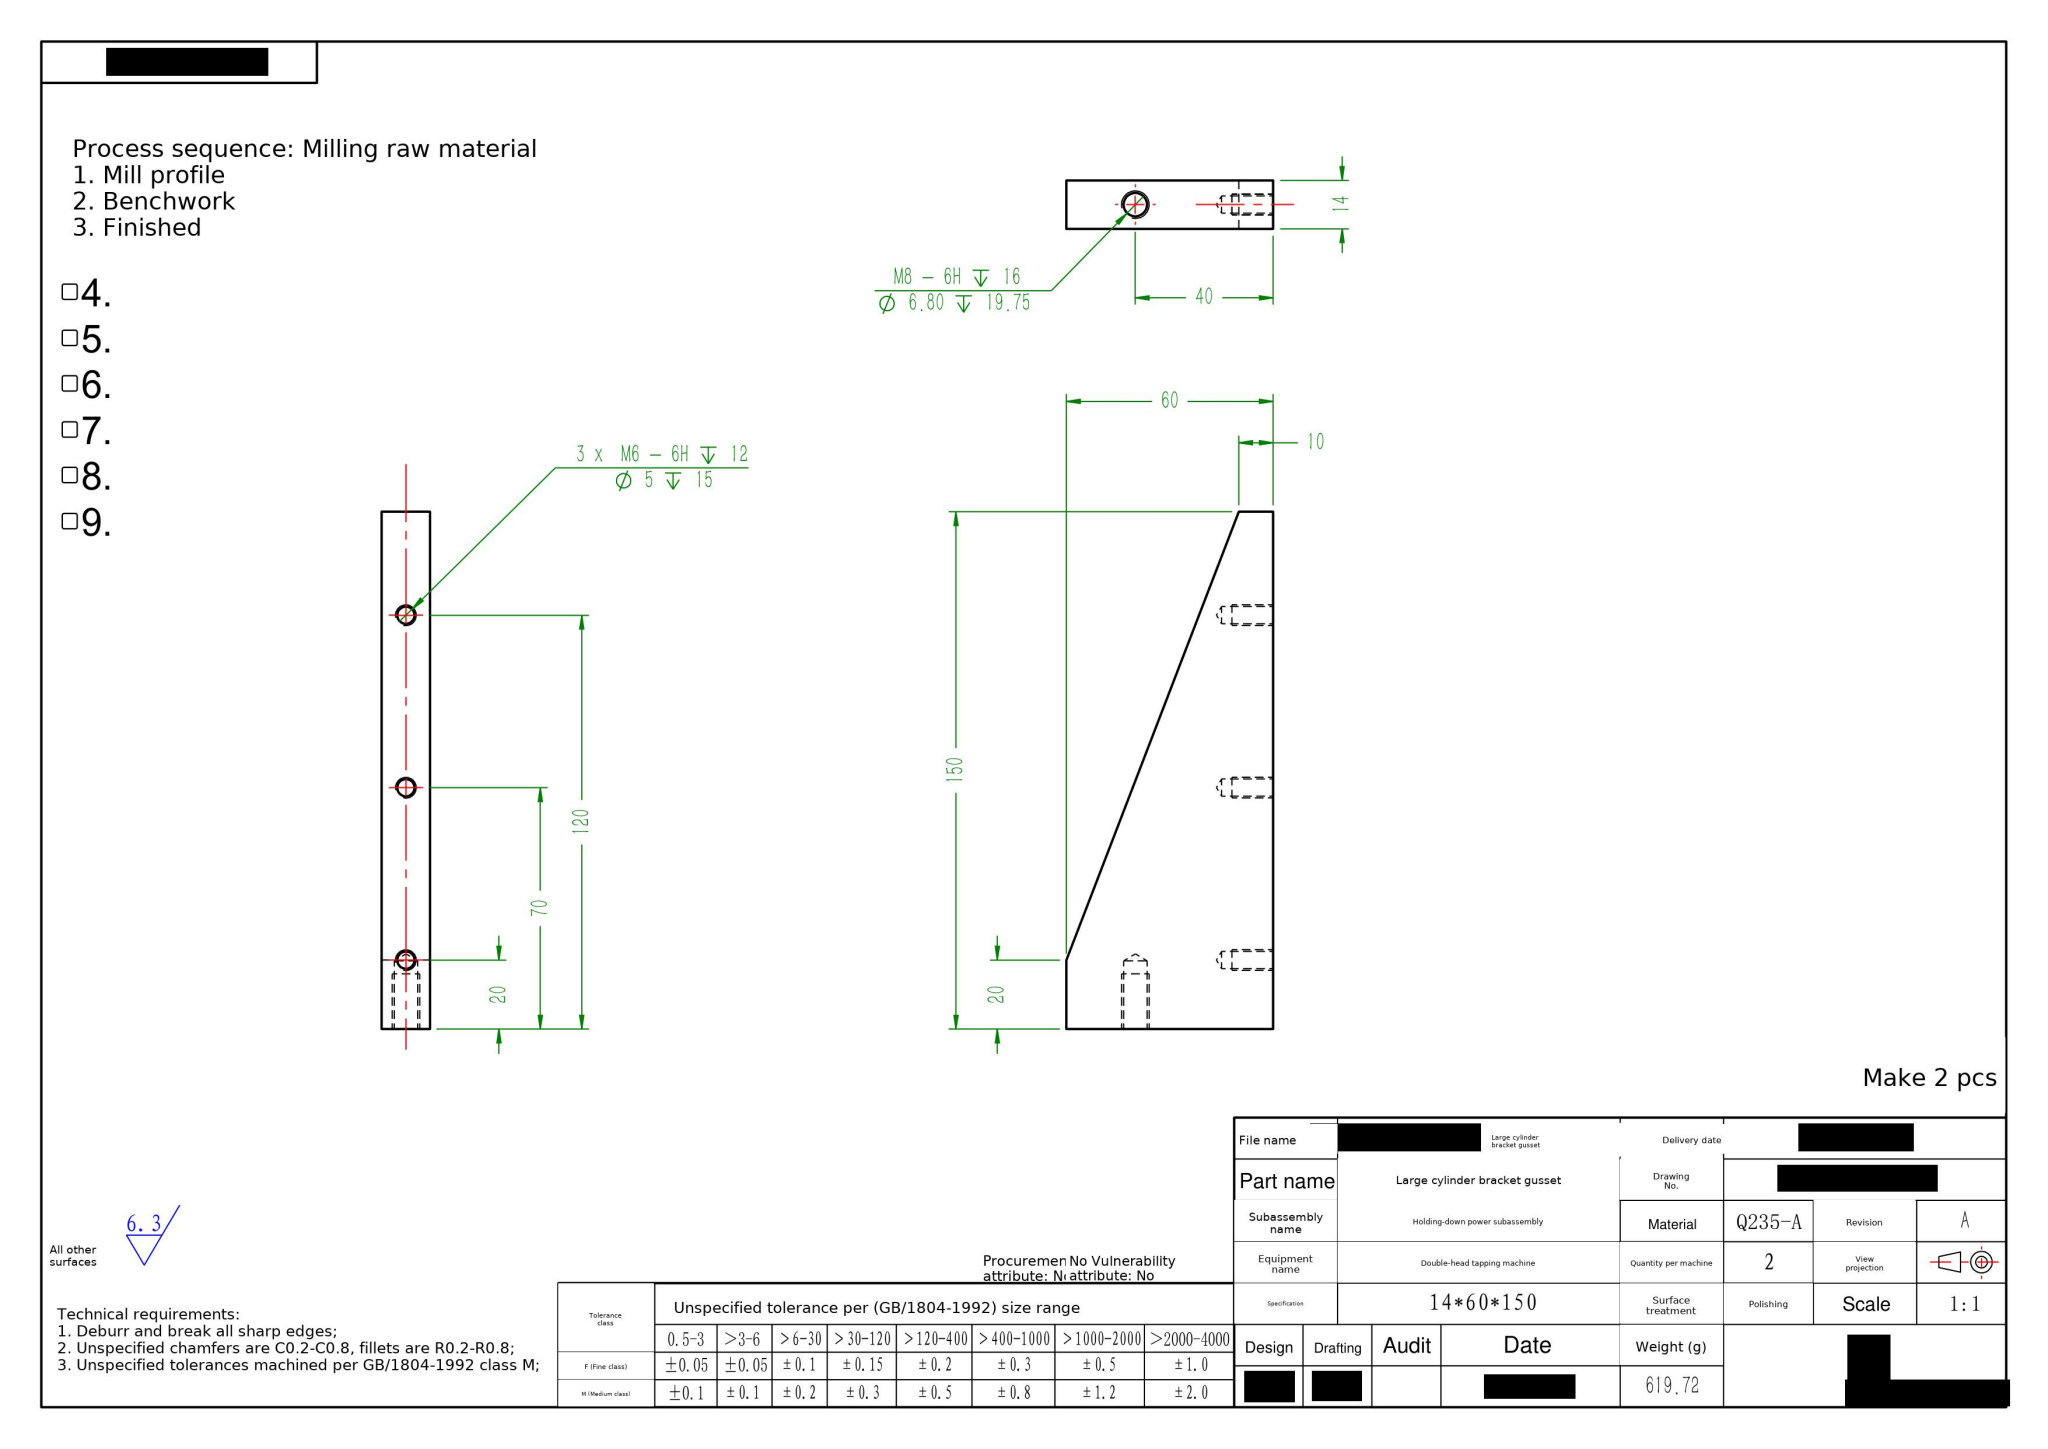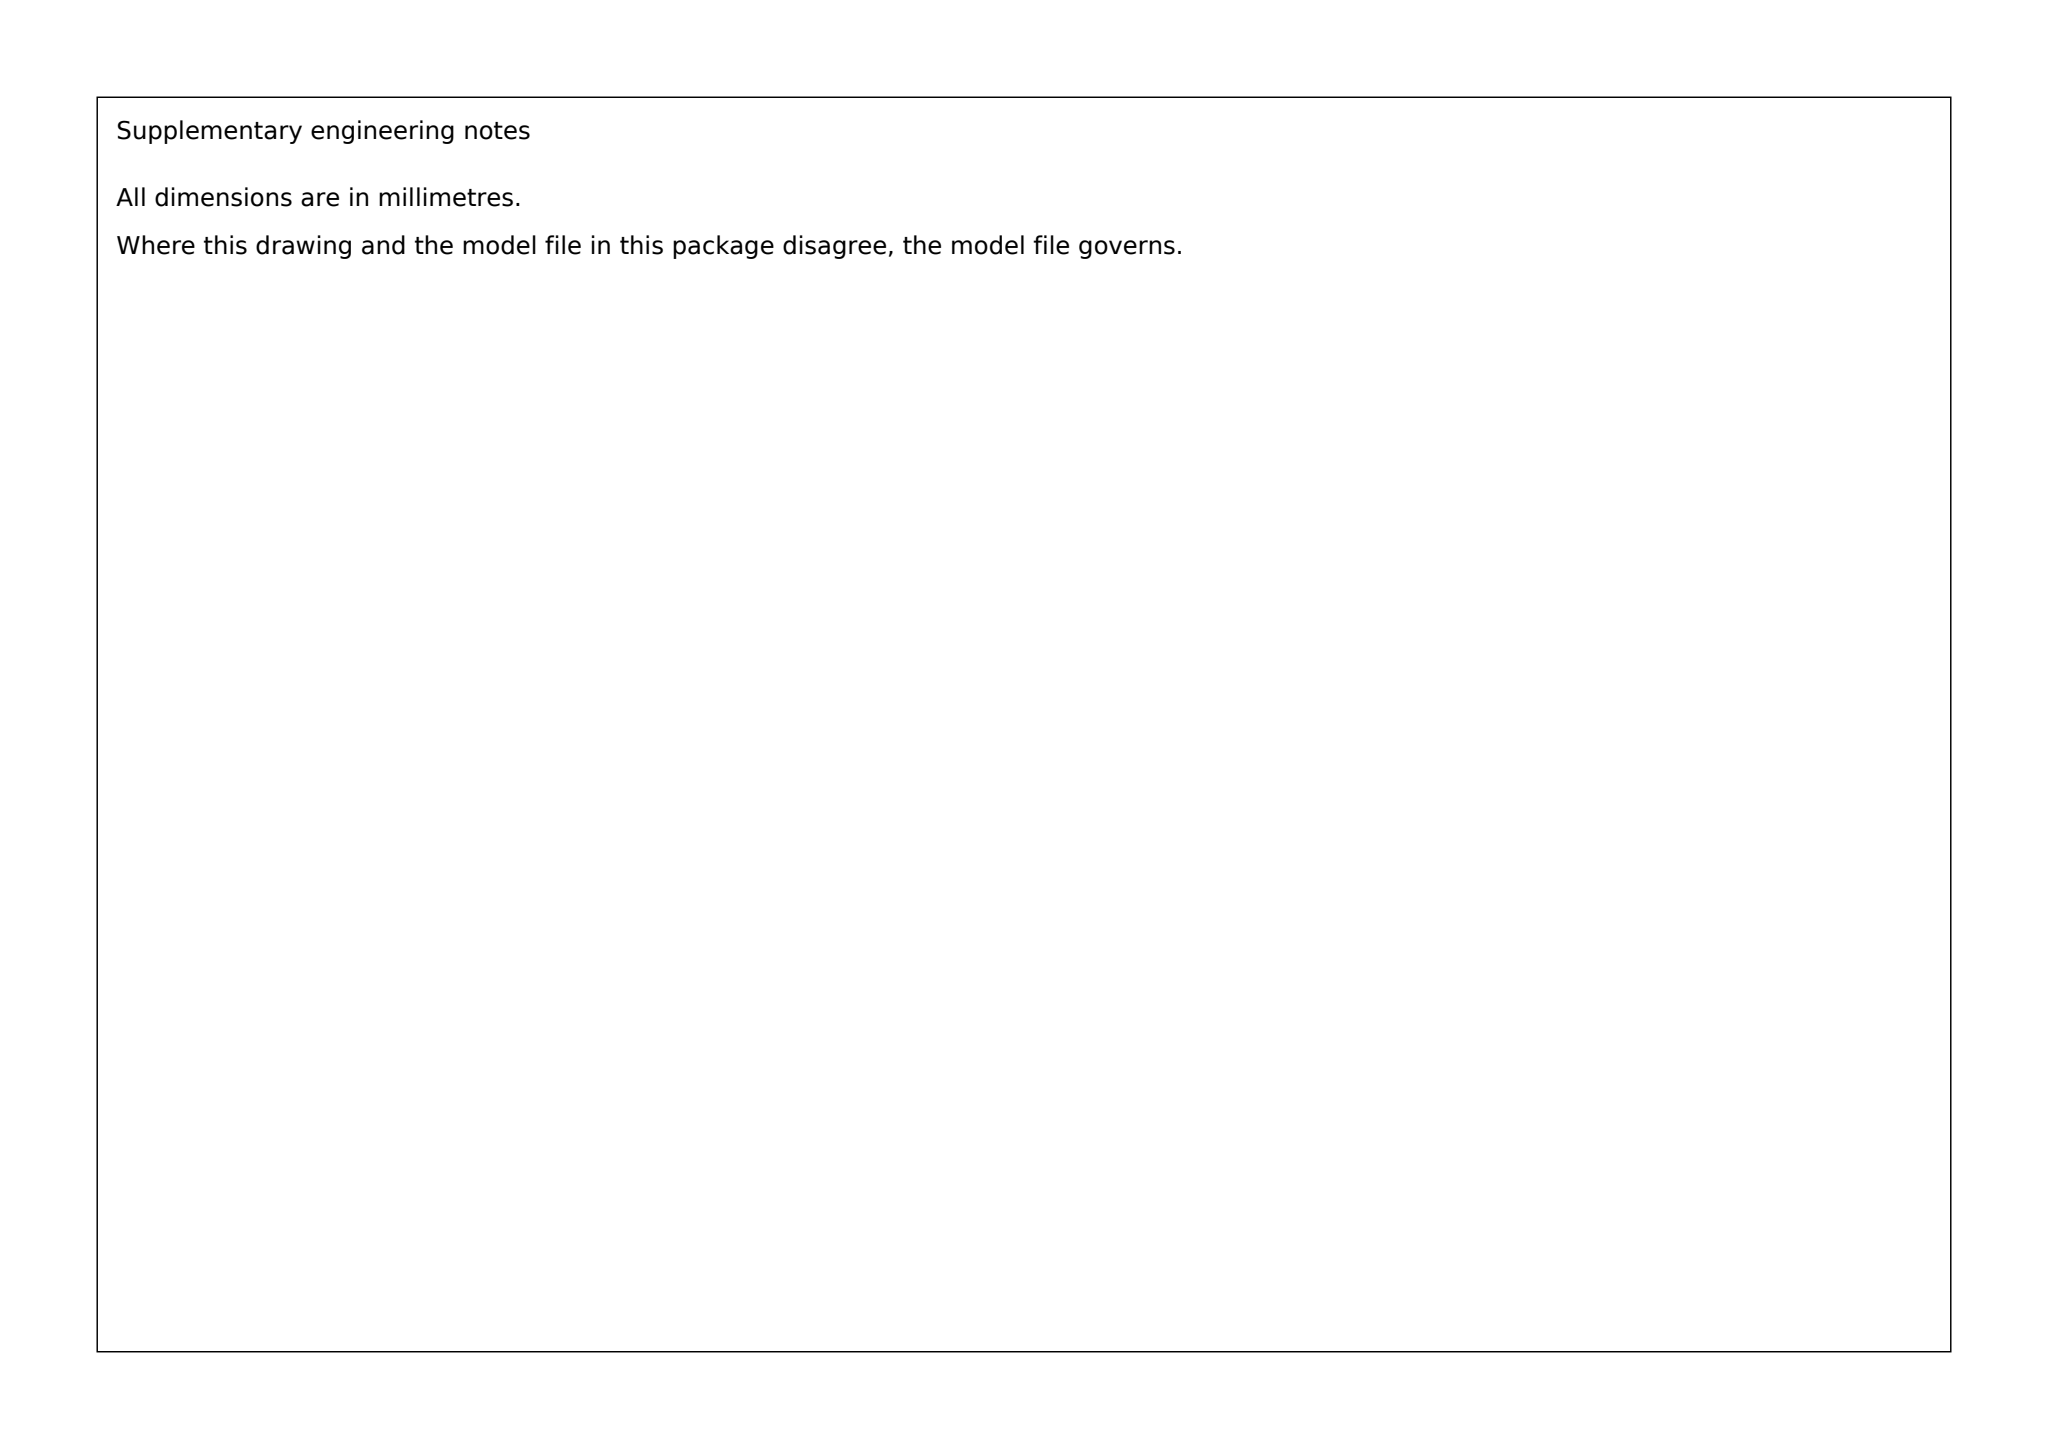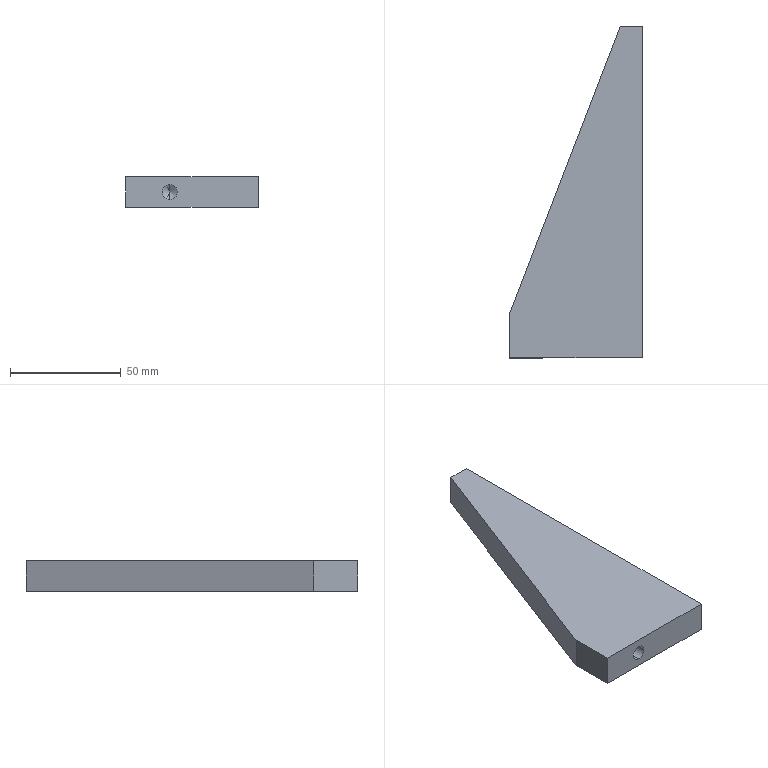Part | SolidWorks | mm | material Q235-A | 1 solid | 23 faces | box 60 x 150 x 14 mm | volume 78845 mm3 | cylinder 8 | cone 8 | plane 7 | commonest cylinder face diameters 5 x6 6.8 x2
build123d program:
from build123d import *

# Parameters (mm, degrees)
BOSS_EXTRUDE1_DEPTH   = 7
M6_TAPPED_HOLE1_D     = 5
M6_TAPPED_HOLE1_DEPTH = 15
M6_TAPPED_HOLE1_TIP   = 1.502
M8_TAPPED_HOLE1_D     = 6.8
M8_TAPPED_HOLE1_DEPTH = 19.75
M8_TAPPED_HOLE1_TIP   = 2.043


with BuildPart() as part:
    # Sketch1 → Boss-Extrude1 (new, symmetric)
    with BuildSketch(Plane.XY):
        Polygon((0, 0), (-60, 0), (-60, 20), (-10, 150), (0, 150), align=None)
    extrude(amount=BOSS_EXTRUDE1_DEPTH, both=True)

    # M6 Tapped Hole1
    with Locations(Plane(origin=(0, 0, 0), x_dir=(0, 0, -1), z_dir=(1, 0, 0))):
        with Locations((0, 20), (0, 70), (0, 120)):
            Hole(M6_TAPPED_HOLE1_D / 2, depth=M6_TAPPED_HOLE1_DEPTH)
            with Locations((0, 0, -(M6_TAPPED_HOLE1_DEPTH + M6_TAPPED_HOLE1_TIP / 2))):  # 118° drill point
                Cone(0, M6_TAPPED_HOLE1_D / 2, M6_TAPPED_HOLE1_TIP, mode=Mode.SUBTRACT)

    # M8 Tapped Hole1
    with Locations(Plane(origin=(0, 0, 0), x_dir=(-1, 0, 0), z_dir=(0, -1, 0))):
        with Locations((40, 0)):
            Hole(M8_TAPPED_HOLE1_D / 2, depth=M8_TAPPED_HOLE1_DEPTH)
            with Locations((0, 0, -(M8_TAPPED_HOLE1_DEPTH + M8_TAPPED_HOLE1_TIP / 2))):  # 118° drill point
                Cone(0, M8_TAPPED_HOLE1_D / 2, M8_TAPPED_HOLE1_TIP, mode=Mode.SUBTRACT)


solid = part.part
STEP:
#1=CARTESIAN_POINT('',(-40.,19.75,3.4));
#2=VERTEX_POINT('',#1);
#3=CARTESIAN_POINT('',(-40.,19.75,-3.4));
#4=VERTEX_POINT('',#3);
#5=CARTESIAN_POINT('',(-40.,19.75,0.));
#6=DIRECTION('',(0.,-1.,0.));
#7=DIRECTION('',(0.,0.,-1.));
#8=AXIS2_PLACEMENT_3D('',#5,#6,#7);
#9=CIRCLE('',#8,3.4);
#10=EDGE_CURVE('',#2,#4,#9,.T.);
#11=ORIENTED_EDGE('',*,*,#10,.F.);
#12=CARTESIAN_POINT('',(-40.,-0.,3.4));
#13=VERTEX_POINT('',#12);
#14=CARTESIAN_POINT('',(-40.,-0.,3.4));
#15=DIRECTION('',(0.,-1.,0.));
#16=VECTOR('',#15,1000.);
#17=LINE('',#14,#16);
#18=EDGE_CURVE('',#2,#13,#17,.T.);
#19=ORIENTED_EDGE('',*,*,#18,.T.);
#20=CARTESIAN_POINT('',(-40.,-0.,-3.4));
#21=VERTEX_POINT('',#20);
#22=CARTESIAN_POINT('',(-40.,-0.,0.));
#23=DIRECTION('',(0.,-1.,0.));
#24=DIRECTION('',(0.,0.,-1.));
#25=AXIS2_PLACEMENT_3D('',#22,#23,#24);
#26=CIRCLE('',#25,3.4);
#27=EDGE_CURVE('',#13,#21,#26,.T.);
#28=ORIENTED_EDGE('',*,*,#27,.T.);
#29=CARTESIAN_POINT('',(-40.,-0.,-3.4));
#30=DIRECTION('',(0.,-1.,0.));
#31=VECTOR('',#30,1000.);
#32=LINE('',#29,#31);
#33=EDGE_CURVE('',#4,#21,#32,.T.);
#34=ORIENTED_EDGE('',*,*,#33,.F.);
#35=EDGE_LOOP('',(#11,#19,#28,#34));
#36=FACE_OUTER_BOUND('',#35,.T.);
#37=CARTESIAN_POINT('',(-40.,-0.,0.));
#38=DIRECTION('',(0.,-1.,0.));
#39=DIRECTION('',(0.,0.,-1.));
#40=AXIS2_PLACEMENT_3D('',#37,#38,#39);
#41=CYLINDRICAL_SURFACE('',#40,3.4);
#42=ADVANCED_FACE('',(#36),#41,.F.);
#43=CARTESIAN_POINT('',(-40.,21.793,0.));
#44=VERTEX_POINT('',#43);
#45=CARTESIAN_POINT('',(-40.,19.75,-3.4));
#46=DIRECTION('',(0.,-0.515,-0.8572));
#47=VECTOR('',#46,1000.);
#48=LINE('',#45,#47);
#49=EDGE_CURVE('',#44,#4,#48,.T.);
#50=ORIENTED_EDGE('',*,*,#49,.F.);
#51=CARTESIAN_POINT('',(-40.,19.75,3.4));
#52=DIRECTION('',(0.,-0.515,0.8572));
#53=VECTOR('',#52,1000.);
#54=LINE('',#51,#53);
#55=EDGE_CURVE('',#44,#2,#54,.T.);
#56=ORIENTED_EDGE('',*,*,#55,.T.);
#57=ORIENTED_EDGE('',*,*,#10,.T.);
#58=EDGE_LOOP('',(#50,#56,#57));
#59=FACE_OUTER_BOUND('',#58,.T.);
#60=CARTESIAN_POINT('',(-40.,19.75,0.));
#61=DIRECTION('',(0.,-1.,0.));
#62=DIRECTION('',(0.,0.,-1.));
#63=AXIS2_PLACEMENT_3D('',#60,#61,#62);
#64=CONICAL_SURFACE('',#63,3.4,1.03);
#65=ADVANCED_FACE('',(#59),#64,.F.);
#66=CARTESIAN_POINT('',(-15.,20.,2.5));
#67=VERTEX_POINT('',#66);
#68=CARTESIAN_POINT('',(-15.,20.,-2.5));
#69=VERTEX_POINT('',#68);
#70=CARTESIAN_POINT('',(-15.,20.,0.));
#71=DIRECTION('',(1.,0.,0.));
#72=DIRECTION('',(0.,0.,-1.));
#73=AXIS2_PLACEMENT_3D('',#70,#71,#72);
#74=CIRCLE('',#73,2.5);
#75=EDGE_CURVE('',#67,#69,#74,.T.);
#76=ORIENTED_EDGE('',*,*,#75,.F.);
#77=CARTESIAN_POINT('',(0.,20.,2.5));
#78=VERTEX_POINT('',#77);
#79=CARTESIAN_POINT('',(0.,20.,2.5));
#80=DIRECTION('',(1.,0.,0.));
#81=VECTOR('',#80,1000.);
#82=LINE('',#79,#81);
#83=EDGE_CURVE('',#67,#78,#82,.T.);
#84=ORIENTED_EDGE('',*,*,#83,.T.);
#85=CARTESIAN_POINT('',(0.,20.,-2.5));
#86=VERTEX_POINT('',#85);
#87=CARTESIAN_POINT('',(0.,20.,0.));
#88=DIRECTION('',(1.,0.,0.));
#89=DIRECTION('',(0.,0.,-1.));
#90=AXIS2_PLACEMENT_3D('',#87,#88,#89);
#91=CIRCLE('',#90,2.5);
#92=EDGE_CURVE('',#78,#86,#91,.T.);
#93=ORIENTED_EDGE('',*,*,#92,.T.);
#94=CARTESIAN_POINT('',(0.,20.,-2.5));
#95=DIRECTION('',(1.,0.,0.));
#96=VECTOR('',#95,1000.);
#97=LINE('',#94,#96);
#98=EDGE_CURVE('',#69,#86,#97,.T.);
#99=ORIENTED_EDGE('',*,*,#98,.F.);
#100=EDGE_LOOP('',(#76,#84,#93,#99));
#101=FACE_OUTER_BOUND('',#100,.T.);
#102=CARTESIAN_POINT('',(0.,20.,0.));
#103=DIRECTION('',(1.,0.,0.));
#104=DIRECTION('',(0.,0.,-1.));
#105=AXIS2_PLACEMENT_3D('',#102,#103,#104);
#106=CYLINDRICAL_SURFACE('',#105,2.5);
#107=ADVANCED_FACE('',(#101),#106,.F.);
#108=CARTESIAN_POINT('',(-16.502,20.,0.));
#109=VERTEX_POINT('',#108);
#110=CARTESIAN_POINT('',(-15.,20.,-2.5));
#111=DIRECTION('',(0.515,0.,-0.8572));
#112=VECTOR('',#111,1000.);
#113=LINE('',#110,#112);
#114=EDGE_CURVE('',#109,#69,#113,.T.);
#115=ORIENTED_EDGE('',*,*,#114,.F.);
#116=CARTESIAN_POINT('',(-15.,20.,2.5));
#117=DIRECTION('',(0.515,0.,0.8572));
#118=VECTOR('',#117,1000.);
#119=LINE('',#116,#118);
#120=EDGE_CURVE('',#109,#67,#119,.T.);
#121=ORIENTED_EDGE('',*,*,#120,.T.);
#122=ORIENTED_EDGE('',*,*,#75,.T.);
#123=EDGE_LOOP('',(#115,#121,#122));
#124=FACE_OUTER_BOUND('',#123,.T.);
#125=CARTESIAN_POINT('',(-15.,20.,0.));
#126=DIRECTION('',(1.,0.,0.));
#127=DIRECTION('',(0.,0.,-1.));
#128=AXIS2_PLACEMENT_3D('',#125,#126,#127);
#129=CONICAL_SURFACE('',#128,2.5,1.03);
#130=ADVANCED_FACE('',(#124),#129,.F.);
#131=CARTESIAN_POINT('',(-15.,70.,2.5));
#132=VERTEX_POINT('',#131);
#133=CARTESIAN_POINT('',(-15.,70.,-2.5));
#134=VERTEX_POINT('',#133);
#135=CARTESIAN_POINT('',(-15.,70.,0.));
#136=DIRECTION('',(1.,0.,0.));
#137=DIRECTION('',(0.,0.,-1.));
#138=AXIS2_PLACEMENT_3D('',#135,#136,#137);
#139=CIRCLE('',#138,2.5);
#140=EDGE_CURVE('',#132,#134,#139,.T.);
#141=ORIENTED_EDGE('',*,*,#140,.F.);
#142=CARTESIAN_POINT('',(0.,70.,2.5));
#143=VERTEX_POINT('',#142);
#144=CARTESIAN_POINT('',(0.,70.,2.5));
#145=DIRECTION('',(1.,0.,0.));
#146=VECTOR('',#145,1000.);
#147=LINE('',#144,#146);
#148=EDGE_CURVE('',#132,#143,#147,.T.);
#149=ORIENTED_EDGE('',*,*,#148,.T.);
#150=CARTESIAN_POINT('',(0.,70.,-2.5));
#151=VERTEX_POINT('',#150);
#152=CARTESIAN_POINT('',(0.,70.,0.));
#153=DIRECTION('',(1.,0.,0.));
#154=DIRECTION('',(0.,0.,-1.));
#155=AXIS2_PLACEMENT_3D('',#152,#153,#154);
#156=CIRCLE('',#155,2.5);
#157=EDGE_CURVE('',#143,#151,#156,.T.);
#158=ORIENTED_EDGE('',*,*,#157,.T.);
#159=CARTESIAN_POINT('',(0.,70.,-2.5));
#160=DIRECTION('',(1.,0.,0.));
#161=VECTOR('',#160,1000.);
#162=LINE('',#159,#161);
#163=EDGE_CURVE('',#134,#151,#162,.T.);
#164=ORIENTED_EDGE('',*,*,#163,.F.);
#165=EDGE_LOOP('',(#141,#149,#158,#164));
#166=FACE_OUTER_BOUND('',#165,.T.);
#167=CARTESIAN_POINT('',(0.,70.,0.));
#168=DIRECTION('',(1.,0.,0.));
#169=DIRECTION('',(0.,0.,-1.));
#170=AXIS2_PLACEMENT_3D('',#167,#168,#169);
#171=CYLINDRICAL_SURFACE('',#170,2.5);
#172=ADVANCED_FACE('',(#166),#171,.F.);
#173=CARTESIAN_POINT('',(-16.502,70.,0.));
#174=VERTEX_POINT('',#173);
#175=CARTESIAN_POINT('',(-15.,70.,-2.5));
#176=DIRECTION('',(0.515,0.,-0.8572));
#177=VECTOR('',#176,1000.);
#178=LINE('',#175,#177);
#179=EDGE_CURVE('',#174,#134,#178,.T.);
#180=ORIENTED_EDGE('',*,*,#179,.F.);
#181=CARTESIAN_POINT('',(-15.,70.,2.5));
#182=DIRECTION('',(0.515,0.,0.8572));
#183=VECTOR('',#182,1000.);
#184=LINE('',#181,#183);
#185=EDGE_CURVE('',#174,#132,#184,.T.);
#186=ORIENTED_EDGE('',*,*,#185,.T.);
#187=ORIENTED_EDGE('',*,*,#140,.T.);
#188=EDGE_LOOP('',(#180,#186,#187));
#189=FACE_OUTER_BOUND('',#188,.T.);
#190=CARTESIAN_POINT('',(-15.,70.,0.));
#191=DIRECTION('',(1.,0.,0.));
#192=DIRECTION('',(0.,0.,-1.));
#193=AXIS2_PLACEMENT_3D('',#190,#191,#192);
#194=CONICAL_SURFACE('',#193,2.5,1.03);
#195=ADVANCED_FACE('',(#189),#194,.F.);
#196=CARTESIAN_POINT('',(-15.,120.,2.5));
#197=VERTEX_POINT('',#196);
#198=CARTESIAN_POINT('',(-15.,120.,-2.5));
#199=VERTEX_POINT('',#198);
#200=CARTESIAN_POINT('',(-15.,120.,0.));
#201=DIRECTION('',(1.,0.,0.));
#202=DIRECTION('',(0.,0.,-1.));
#203=AXIS2_PLACEMENT_3D('',#200,#201,#202);
#204=CIRCLE('',#203,2.5);
#205=EDGE_CURVE('',#197,#199,#204,.T.);
#206=ORIENTED_EDGE('',*,*,#205,.F.);
#207=CARTESIAN_POINT('',(0.,120.,2.5));
#208=VERTEX_POINT('',#207);
#209=CARTESIAN_POINT('',(0.,120.,2.5));
#210=DIRECTION('',(1.,0.,0.));
#211=VECTOR('',#210,1000.);
#212=LINE('',#209,#211);
#213=EDGE_CURVE('',#197,#208,#212,.T.);
#214=ORIENTED_EDGE('',*,*,#213,.T.);
#215=CARTESIAN_POINT('',(0.,120.,-2.5));
#216=VERTEX_POINT('',#215);
#217=CARTESIAN_POINT('',(0.,120.,0.));
#218=DIRECTION('',(1.,0.,0.));
#219=DIRECTION('',(0.,0.,-1.));
#220=AXIS2_PLACEMENT_3D('',#217,#218,#219);
#221=CIRCLE('',#220,2.5);
#222=EDGE_CURVE('',#208,#216,#221,.T.);
#223=ORIENTED_EDGE('',*,*,#222,.T.);
#224=CARTESIAN_POINT('',(0.,120.,-2.5));
#225=DIRECTION('',(1.,0.,0.));
#226=VECTOR('',#225,1000.);
#227=LINE('',#224,#226);
#228=EDGE_CURVE('',#199,#216,#227,.T.);
#229=ORIENTED_EDGE('',*,*,#228,.F.);
#230=EDGE_LOOP('',(#206,#214,#223,#229));
#231=FACE_OUTER_BOUND('',#230,.T.);
#232=CARTESIAN_POINT('',(0.,120.,0.));
#233=DIRECTION('',(1.,0.,0.));
#234=DIRECTION('',(0.,0.,-1.));
#235=AXIS2_PLACEMENT_3D('',#232,#233,#234);
#236=CYLINDRICAL_SURFACE('',#235,2.5);
#237=ADVANCED_FACE('',(#231),#236,.F.);
#238=CARTESIAN_POINT('',(-16.502,120.,0.));
#239=VERTEX_POINT('',#238);
#240=CARTESIAN_POINT('',(-15.,120.,-2.5));
#241=DIRECTION('',(0.515,0.,-0.8572));
#242=VECTOR('',#241,1000.);
#243=LINE('',#240,#242);
#244=EDGE_CURVE('',#239,#199,#243,.T.);
#245=ORIENTED_EDGE('',*,*,#244,.F.);
#246=CARTESIAN_POINT('',(-15.,120.,2.5));
#247=DIRECTION('',(0.515,0.,0.8572));
#248=VECTOR('',#247,1000.);
#249=LINE('',#246,#248);
#250=EDGE_CURVE('',#239,#197,#249,.T.);
#251=ORIENTED_EDGE('',*,*,#250,.T.);
#252=ORIENTED_EDGE('',*,*,#205,.T.);
#253=EDGE_LOOP('',(#245,#251,#252));
#254=FACE_OUTER_BOUND('',#253,.T.);
#255=CARTESIAN_POINT('',(-15.,120.,0.));
#256=DIRECTION('',(1.,0.,0.));
#257=DIRECTION('',(0.,0.,-1.));
#258=AXIS2_PLACEMENT_3D('',#255,#256,#257);
#259=CONICAL_SURFACE('',#258,2.5,1.03);
#260=ADVANCED_FACE('',(#254),#259,.F.);
#261=CARTESIAN_POINT('',(0.,20.,0.));
#262=DIRECTION('',(1.,0.,0.));
#263=DIRECTION('',(0.,0.,-1.));
#264=AXIS2_PLACEMENT_3D('',#261,#262,#263);
#265=CIRCLE('',#264,2.5);
#266=EDGE_CURVE('',#86,#78,#265,.T.);
#267=ORIENTED_EDGE('',*,*,#266,.F.);
#268=ORIENTED_EDGE('',*,*,#92,.F.);
#269=EDGE_LOOP('',(#267,#268));
#270=FACE_BOUND('',#269,.T.);
#271=CARTESIAN_POINT('',(0.,70.,0.));
#272=DIRECTION('',(1.,0.,0.));
#273=DIRECTION('',(0.,0.,-1.));
#274=AXIS2_PLACEMENT_3D('',#271,#272,#273);
#275=CIRCLE('',#274,2.5);
#276=EDGE_CURVE('',#151,#143,#275,.T.);
#277=ORIENTED_EDGE('',*,*,#276,.F.);
#278=ORIENTED_EDGE('',*,*,#157,.F.);
#279=EDGE_LOOP('',(#277,#278));
#280=FACE_BOUND('',#279,.T.);
#281=CARTESIAN_POINT('',(0.,120.,0.));
#282=DIRECTION('',(1.,0.,0.));
#283=DIRECTION('',(0.,0.,-1.));
#284=AXIS2_PLACEMENT_3D('',#281,#282,#283);
#285=CIRCLE('',#284,2.5);
#286=EDGE_CURVE('',#216,#208,#285,.T.);
#287=ORIENTED_EDGE('',*,*,#286,.F.);
#288=ORIENTED_EDGE('',*,*,#222,.F.);
#289=EDGE_LOOP('',(#287,#288));
#290=FACE_BOUND('',#289,.T.);
#291=CARTESIAN_POINT('',(0.,0.,-7.));
#292=VERTEX_POINT('',#291);
#293=CARTESIAN_POINT('',(0.,150.,-7.));
#294=VERTEX_POINT('',#293);
#295=CARTESIAN_POINT('',(0.,150.,-7.));
#296=DIRECTION('',(0.,1.,0.));
#297=VECTOR('',#296,1000.);
#298=LINE('',#295,#297);
#299=EDGE_CURVE('',#292,#294,#298,.T.);
#300=ORIENTED_EDGE('',*,*,#299,.T.);
#301=CARTESIAN_POINT('',(0.,150.,7.));
#302=VERTEX_POINT('',#301);
#303=CARTESIAN_POINT('',(0.,150.,7.));
#304=DIRECTION('',(0.,0.,-1.));
#305=VECTOR('',#304,1000.);
#306=LINE('',#303,#305);
#307=EDGE_CURVE('',#302,#294,#306,.T.);
#308=ORIENTED_EDGE('',*,*,#307,.F.);
#309=CARTESIAN_POINT('',(0.,0.,7.));
#310=VERTEX_POINT('',#309);
#311=CARTESIAN_POINT('',(0.,150.,7.));
#312=DIRECTION('',(0.,1.,0.));
#313=VECTOR('',#312,1000.);
#314=LINE('',#311,#313);
#315=EDGE_CURVE('',#310,#302,#314,.T.);
#316=ORIENTED_EDGE('',*,*,#315,.F.);
#317=CARTESIAN_POINT('',(0.,0.,7.));
#318=DIRECTION('',(0.,0.,-1.));
#319=VECTOR('',#318,1000.);
#320=LINE('',#317,#319);
#321=EDGE_CURVE('',#310,#292,#320,.T.);
#322=ORIENTED_EDGE('',*,*,#321,.T.);
#323=EDGE_LOOP('',(#300,#308,#316,#322));
#324=FACE_OUTER_BOUND('',#323,.T.);
#325=CARTESIAN_POINT('',(0.,150.,7.));
#326=DIRECTION('',(-1.,0.,0.));
#327=DIRECTION('',(0.,0.,1.));
#328=AXIS2_PLACEMENT_3D('',#325,#326,#327);
#329=PLANE('',#328);
#330=ADVANCED_FACE('',(#270,#280,#290,#324),#329,.F.);
#331=CARTESIAN_POINT('',(-10.,150.,-7.));
#332=VERTEX_POINT('',#331);
#333=CARTESIAN_POINT('',(-10.,150.,-7.));
#334=DIRECTION('',(-1.,0.,0.));
#335=VECTOR('',#334,1000.);
#336=LINE('',#333,#335);
#337=EDGE_CURVE('',#294,#332,#336,.T.);
#338=ORIENTED_EDGE('',*,*,#337,.T.);
#339=CARTESIAN_POINT('',(-10.,150.,7.));
#340=VERTEX_POINT('',#339);
#341=CARTESIAN_POINT('',(-10.,150.,7.));
#342=DIRECTION('',(0.,0.,-1.));
#343=VECTOR('',#342,1000.);
#344=LINE('',#341,#343);
#345=EDGE_CURVE('',#340,#332,#344,.T.);
#346=ORIENTED_EDGE('',*,*,#345,.F.);
#347=CARTESIAN_POINT('',(-10.,150.,7.));
#348=DIRECTION('',(-1.,0.,0.));
#349=VECTOR('',#348,1000.);
#350=LINE('',#347,#349);
#351=EDGE_CURVE('',#302,#340,#350,.T.);
#352=ORIENTED_EDGE('',*,*,#351,.F.);
#353=ORIENTED_EDGE('',*,*,#307,.T.);
#354=EDGE_LOOP('',(#338,#346,#352,#353));
#355=FACE_OUTER_BOUND('',#354,.T.);
#356=CARTESIAN_POINT('',(-10.,150.,7.));
#357=DIRECTION('',(0.,-1.,0.));
#358=DIRECTION('',(0.,0.,-1.));
#359=AXIS2_PLACEMENT_3D('',#356,#357,#358);
#360=PLANE('',#359);
#361=ADVANCED_FACE('',(#355),#360,.F.);
#362=CARTESIAN_POINT('',(-60.,20.,-7.));
#363=VERTEX_POINT('',#362);
#364=CARTESIAN_POINT('',(-60.,20.,-7.));
#365=DIRECTION('',(-0.359,-0.9333,0.));
#366=VECTOR('',#365,1000.);
#367=LINE('',#364,#366);
#368=EDGE_CURVE('',#332,#363,#367,.T.);
#369=ORIENTED_EDGE('',*,*,#368,.T.);
#370=CARTESIAN_POINT('',(-60.,20.,7.));
#371=VERTEX_POINT('',#370);
#372=CARTESIAN_POINT('',(-60.,20.,7.));
#373=DIRECTION('',(0.,0.,-1.));
#374=VECTOR('',#373,1000.);
#375=LINE('',#372,#374);
#376=EDGE_CURVE('',#371,#363,#375,.T.);
#377=ORIENTED_EDGE('',*,*,#376,.F.);
#378=CARTESIAN_POINT('',(-60.,20.,7.));
#379=DIRECTION('',(-0.359,-0.9333,0.));
#380=VECTOR('',#379,1000.);
#381=LINE('',#378,#380);
#382=EDGE_CURVE('',#340,#371,#381,.T.);
#383=ORIENTED_EDGE('',*,*,#382,.F.);
#384=ORIENTED_EDGE('',*,*,#345,.T.);
#385=EDGE_LOOP('',(#369,#377,#383,#384));
#386=FACE_OUTER_BOUND('',#385,.T.);
#387=CARTESIAN_POINT('',(-60.,20.,7.));
#388=DIRECTION('',(0.9333,-0.359,0.));
#389=DIRECTION('',(0.359,0.9333,0.));
#390=AXIS2_PLACEMENT_3D('',#387,#388,#389);
#391=PLANE('',#390);
#392=ADVANCED_FACE('',(#386),#391,.F.);
#393=CARTESIAN_POINT('',(-60.,-0.,-7.));
#394=VERTEX_POINT('',#393);
#395=CARTESIAN_POINT('',(-60.,-0.,-7.));
#396=DIRECTION('',(0.,-1.,0.));
#397=VECTOR('',#396,1000.);
#398=LINE('',#395,#397);
#399=EDGE_CURVE('',#363,#394,#398,.T.);
#400=ORIENTED_EDGE('',*,*,#399,.T.);
#401=CARTESIAN_POINT('',(-60.,-0.,7.));
#402=VERTEX_POINT('',#401);
#403=CARTESIAN_POINT('',(-60.,-0.,7.));
#404=DIRECTION('',(0.,0.,-1.));
#405=VECTOR('',#404,1000.);
#406=LINE('',#403,#405);
#407=EDGE_CURVE('',#402,#394,#406,.T.);
#408=ORIENTED_EDGE('',*,*,#407,.F.);
#409=CARTESIAN_POINT('',(-60.,-0.,7.));
#410=DIRECTION('',(0.,-1.,0.));
#411=VECTOR('',#410,1000.);
#412=LINE('',#409,#411);
#413=EDGE_CURVE('',#371,#402,#412,.T.);
#414=ORIENTED_EDGE('',*,*,#413,.F.);
#415=ORIENTED_EDGE('',*,*,#376,.T.);
#416=EDGE_LOOP('',(#400,#408,#414,#415));
#417=FACE_OUTER_BOUND('',#416,.T.);
#418=CARTESIAN_POINT('',(-60.,-0.,7.));
#419=DIRECTION('',(1.,0.,0.));
#420=DIRECTION('',(0.,0.,-1.));
#421=AXIS2_PLACEMENT_3D('',#418,#419,#420);
#422=PLANE('',#421);
#423=ADVANCED_FACE('',(#417),#422,.F.);
#424=CARTESIAN_POINT('',(-40.,-0.,0.));
#425=DIRECTION('',(0.,-1.,0.));
#426=DIRECTION('',(0.,0.,-1.));
#427=AXIS2_PLACEMENT_3D('',#424,#425,#426);
#428=CIRCLE('',#427,3.4);
#429=EDGE_CURVE('',#21,#13,#428,.T.);
#430=ORIENTED_EDGE('',*,*,#429,.F.);
#431=ORIENTED_EDGE('',*,*,#27,.F.);
#432=EDGE_LOOP('',(#430,#431));
#433=FACE_BOUND('',#432,.T.);
#434=CARTESIAN_POINT('',(0.,0.,-7.));
#435=DIRECTION('',(1.,0.,0.));
#436=VECTOR('',#435,1000.);
#437=LINE('',#434,#436);
#438=EDGE_CURVE('',#394,#292,#437,.T.);
#439=ORIENTED_EDGE('',*,*,#438,.T.);
#440=ORIENTED_EDGE('',*,*,#321,.F.);
#441=CARTESIAN_POINT('',(0.,0.,7.));
#442=DIRECTION('',(1.,0.,0.));
#443=VECTOR('',#442,1000.);
#444=LINE('',#441,#443);
#445=EDGE_CURVE('',#402,#310,#444,.T.);
#446=ORIENTED_EDGE('',*,*,#445,.F.);
#447=ORIENTED_EDGE('',*,*,#407,.T.);
#448=EDGE_LOOP('',(#439,#440,#446,#447));
#449=FACE_OUTER_BOUND('',#448,.T.);
#450=CARTESIAN_POINT('',(0.,0.,7.));
#451=DIRECTION('',(-0.,1.,0.));
#452=DIRECTION('',(-1.,-0.,0.));
#453=AXIS2_PLACEMENT_3D('',#450,#451,#452);
#454=PLANE('',#453);
#455=ADVANCED_FACE('',(#433,#449),#454,.F.);
#456=ORIENTED_EDGE('',*,*,#315,.T.);
#457=ORIENTED_EDGE('',*,*,#351,.T.);
#458=ORIENTED_EDGE('',*,*,#382,.T.);
#459=ORIENTED_EDGE('',*,*,#413,.T.);
#460=ORIENTED_EDGE('',*,*,#445,.T.);
#461=EDGE_LOOP('',(#456,#457,#458,#459,#460));
#462=FACE_OUTER_BOUND('',#461,.T.);
#463=CARTESIAN_POINT('',(0.,0.,7.));
#464=DIRECTION('',(0.,0.,-1.));
#465=DIRECTION('',(-1.,0.,0.));
#466=AXIS2_PLACEMENT_3D('',#463,#464,#465);
#467=PLANE('',#466);
#468=ADVANCED_FACE('',(#462),#467,.F.);
#469=ORIENTED_EDGE('',*,*,#299,.F.);
#470=ORIENTED_EDGE('',*,*,#438,.F.);
#471=ORIENTED_EDGE('',*,*,#399,.F.);
#472=ORIENTED_EDGE('',*,*,#368,.F.);
#473=ORIENTED_EDGE('',*,*,#337,.F.);
#474=EDGE_LOOP('',(#469,#470,#471,#472,#473));
#475=FACE_OUTER_BOUND('',#474,.T.);
#476=CARTESIAN_POINT('',(0.,0.,-7.));
#477=DIRECTION('',(0.,0.,-1.));
#478=DIRECTION('',(-1.,0.,0.));
#479=AXIS2_PLACEMENT_3D('',#476,#477,#478);
#480=PLANE('',#479);
#481=ADVANCED_FACE('',(#475),#480,.T.);
#482=ORIENTED_EDGE('',*,*,#250,.F.);
#483=ORIENTED_EDGE('',*,*,#244,.T.);
#484=CARTESIAN_POINT('',(-15.,120.,0.));
#485=DIRECTION('',(1.,0.,0.));
#486=DIRECTION('',(0.,0.,-1.));
#487=AXIS2_PLACEMENT_3D('',#484,#485,#486);
#488=CIRCLE('',#487,2.5);
#489=EDGE_CURVE('',#199,#197,#488,.T.);
#490=ORIENTED_EDGE('',*,*,#489,.T.);
#491=EDGE_LOOP('',(#482,#483,#490));
#492=FACE_OUTER_BOUND('',#491,.T.);
#493=CARTESIAN_POINT('',(-15.,120.,0.));
#494=DIRECTION('',(1.,0.,0.));
#495=DIRECTION('',(0.,0.,-1.));
#496=AXIS2_PLACEMENT_3D('',#493,#494,#495);
#497=CONICAL_SURFACE('',#496,2.5,1.03);
#498=ADVANCED_FACE('',(#492),#497,.F.);
#499=ORIENTED_EDGE('',*,*,#213,.F.);
#500=ORIENTED_EDGE('',*,*,#489,.F.);
#501=ORIENTED_EDGE('',*,*,#228,.T.);
#502=ORIENTED_EDGE('',*,*,#286,.T.);
#503=EDGE_LOOP('',(#499,#500,#501,#502));
#504=FACE_OUTER_BOUND('',#503,.T.);
#505=CARTESIAN_POINT('',(0.,120.,0.));
#506=DIRECTION('',(1.,0.,0.));
#507=DIRECTION('',(0.,0.,-1.));
#508=AXIS2_PLACEMENT_3D('',#505,#506,#507);
#509=CYLINDRICAL_SURFACE('',#508,2.5);
#510=ADVANCED_FACE('',(#504),#509,.F.);
#511=ORIENTED_EDGE('',*,*,#185,.F.);
#512=ORIENTED_EDGE('',*,*,#179,.T.);
#513=CARTESIAN_POINT('',(-15.,70.,0.));
#514=DIRECTION('',(1.,0.,0.));
#515=DIRECTION('',(0.,0.,-1.));
#516=AXIS2_PLACEMENT_3D('',#513,#514,#515);
#517=CIRCLE('',#516,2.5);
#518=EDGE_CURVE('',#134,#132,#517,.T.);
#519=ORIENTED_EDGE('',*,*,#518,.T.);
#520=EDGE_LOOP('',(#511,#512,#519));
#521=FACE_OUTER_BOUND('',#520,.T.);
#522=CARTESIAN_POINT('',(-15.,70.,0.));
#523=DIRECTION('',(1.,0.,0.));
#524=DIRECTION('',(0.,0.,-1.));
#525=AXIS2_PLACEMENT_3D('',#522,#523,#524);
#526=CONICAL_SURFACE('',#525,2.5,1.03);
#527=ADVANCED_FACE('',(#521),#526,.F.);
#528=ORIENTED_EDGE('',*,*,#148,.F.);
#529=ORIENTED_EDGE('',*,*,#518,.F.);
#530=ORIENTED_EDGE('',*,*,#163,.T.);
#531=ORIENTED_EDGE('',*,*,#276,.T.);
#532=EDGE_LOOP('',(#528,#529,#530,#531));
#533=FACE_OUTER_BOUND('',#532,.T.);
#534=CARTESIAN_POINT('',(0.,70.,0.));
#535=DIRECTION('',(1.,0.,0.));
#536=DIRECTION('',(0.,0.,-1.));
#537=AXIS2_PLACEMENT_3D('',#534,#535,#536);
#538=CYLINDRICAL_SURFACE('',#537,2.5);
#539=ADVANCED_FACE('',(#533),#538,.F.);
#540=ORIENTED_EDGE('',*,*,#120,.F.);
#541=ORIENTED_EDGE('',*,*,#114,.T.);
#542=CARTESIAN_POINT('',(-15.,20.,0.));
#543=DIRECTION('',(1.,0.,0.));
#544=DIRECTION('',(0.,0.,-1.));
#545=AXIS2_PLACEMENT_3D('',#542,#543,#544);
#546=CIRCLE('',#545,2.5);
#547=EDGE_CURVE('',#69,#67,#546,.T.);
#548=ORIENTED_EDGE('',*,*,#547,.T.);
#549=EDGE_LOOP('',(#540,#541,#548));
#550=FACE_OUTER_BOUND('',#549,.T.);
#551=CARTESIAN_POINT('',(-15.,20.,0.));
#552=DIRECTION('',(1.,0.,0.));
#553=DIRECTION('',(0.,0.,-1.));
#554=AXIS2_PLACEMENT_3D('',#551,#552,#553);
#555=CONICAL_SURFACE('',#554,2.5,1.03);
#556=ADVANCED_FACE('',(#550),#555,.F.);
#557=ORIENTED_EDGE('',*,*,#83,.F.);
#558=ORIENTED_EDGE('',*,*,#547,.F.);
#559=ORIENTED_EDGE('',*,*,#98,.T.);
#560=ORIENTED_EDGE('',*,*,#266,.T.);
#561=EDGE_LOOP('',(#557,#558,#559,#560));
#562=FACE_OUTER_BOUND('',#561,.T.);
#563=CARTESIAN_POINT('',(0.,20.,0.));
#564=DIRECTION('',(1.,0.,0.));
#565=DIRECTION('',(0.,0.,-1.));
#566=AXIS2_PLACEMENT_3D('',#563,#564,#565);
#567=CYLINDRICAL_SURFACE('',#566,2.5);
#568=ADVANCED_FACE('',(#562),#567,.F.);
#569=ORIENTED_EDGE('',*,*,#55,.F.);
#570=ORIENTED_EDGE('',*,*,#49,.T.);
#571=CARTESIAN_POINT('',(-40.,19.75,0.));
#572=DIRECTION('',(0.,-1.,0.));
#573=DIRECTION('',(0.,0.,-1.));
#574=AXIS2_PLACEMENT_3D('',#571,#572,#573);
#575=CIRCLE('',#574,3.4);
#576=EDGE_CURVE('',#4,#2,#575,.T.);
#577=ORIENTED_EDGE('',*,*,#576,.T.);
#578=EDGE_LOOP('',(#569,#570,#577));
#579=FACE_OUTER_BOUND('',#578,.T.);
#580=CARTESIAN_POINT('',(-40.,19.75,0.));
#581=DIRECTION('',(0.,-1.,0.));
#582=DIRECTION('',(0.,0.,-1.));
#583=AXIS2_PLACEMENT_3D('',#580,#581,#582);
#584=CONICAL_SURFACE('',#583,3.4,1.03);
#585=ADVANCED_FACE('',(#579),#584,.F.);
#586=ORIENTED_EDGE('',*,*,#18,.F.);
#587=ORIENTED_EDGE('',*,*,#576,.F.);
#588=ORIENTED_EDGE('',*,*,#33,.T.);
#589=ORIENTED_EDGE('',*,*,#429,.T.);
#590=EDGE_LOOP('',(#586,#587,#588,#589));
#591=FACE_OUTER_BOUND('',#590,.T.);
#592=CARTESIAN_POINT('',(-40.,-0.,0.));
#593=DIRECTION('',(0.,-1.,0.));
#594=DIRECTION('',(0.,0.,-1.));
#595=AXIS2_PLACEMENT_3D('',#592,#593,#594);
#596=CYLINDRICAL_SURFACE('',#595,3.4);
#597=ADVANCED_FACE('',(#591),#596,.F.);
#598=CLOSED_SHELL('',(#42,#65,#107,#130,#172,#195,#237,#260,#330,#361,#392,#423,#455,#468,#481,#498,#510,#527,#539,#556,#568,#585,#597));
#599=MANIFOLD_SOLID_BREP('',#598);
#600=CARTESIAN_POINT('',(0.,0.,0.));
#601=DIRECTION('',(0.,0.,1.));
#602=DIRECTION('',(1.,0.,0.));
#603=AXIS2_PLACEMENT_3D('',#600,#601,#602);
#604=(LENGTH_UNIT()NAMED_UNIT(*)SI_UNIT(.MILLI.,.METRE.));
#605=UNCERTAINTY_MEASURE_WITH_UNIT(LENGTH_MEASURE(0.00001),#604,'','');
#606=(NAMED_UNIT(*)PLANE_ANGLE_UNIT()SI_UNIT($,.RADIAN.));
#607=(NAMED_UNIT(*)SI_UNIT($,.STERADIAN.)SOLID_ANGLE_UNIT());
#608=(GEOMETRIC_REPRESENTATION_CONTEXT(3)GLOBAL_UNCERTAINTY_ASSIGNED_CONTEXT((#605))GLOBAL_UNIT_ASSIGNED_CONTEXT((#604,#606,#607))REPRESENTATION_CONTEXT('',''));
#609=ADVANCED_BREP_SHAPE_REPRESENTATION('',(#599,#603),#608);